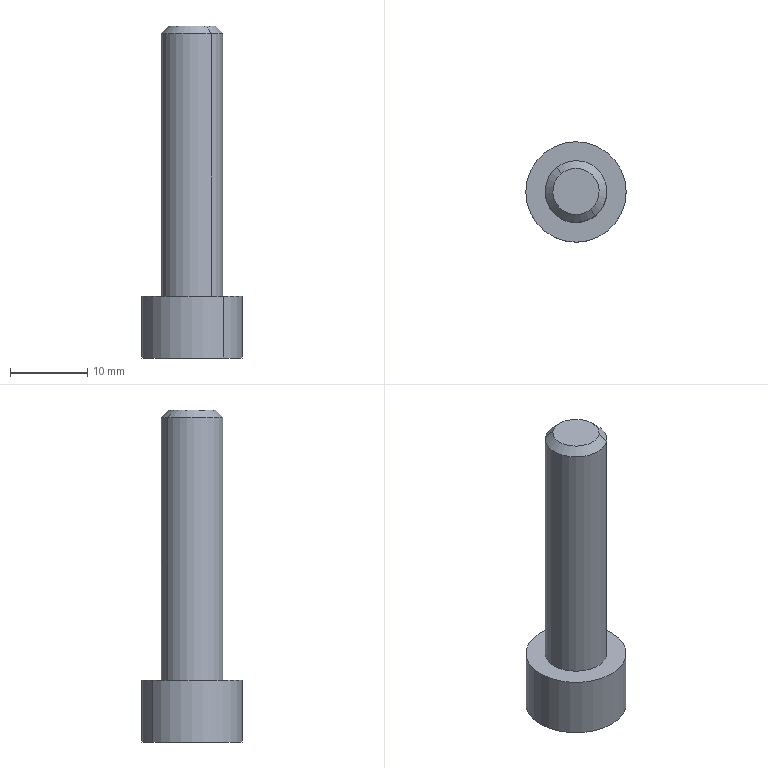Component | SolidWorks | 9HexSocketScrewM8X35-1 | 1 solid | 23 faces | box 13 x 13 x 43 mm | volume 2614 mm3 | plane 15 | cone 4 | cylinder 4 | commonest cylinder face diameters 8 x2 13 x2
STEP:
#1=CARTESIAN_POINT('',(1.263,2.918,7.047));
#2=VERTEX_POINT('',#1);
#3=CARTESIAN_POINT('',(1.411,2.734,7.047));
#4=VERTEX_POINT('',#3);
#5=CARTESIAN_POINT('',(1.337,2.826,7.047));
#6=DIRECTION('',(-0.,-0.,1.));
#7=DIRECTION('',(-0.6242,0.7813,0.));
#8=AXIS2_PLACEMENT_3D('',#5,#6,#7);
#9=CIRCLE('',#8,0.1181);
#10=EDGE_CURVE('',#2,#4,#9,.T.);
#11=ORIENTED_EDGE('',*,*,#10,.F.);
#12=CARTESIAN_POINT('',(1.239,2.949,7.008));
#13=VERTEX_POINT('',#12);
#14=CARTESIAN_POINT('',(1.263,2.918,7.047));
#15=DIRECTION('',(-0.4414,0.5524,-0.7071));
#16=VECTOR('',#15,39.37);
#17=LINE('',#14,#16);
#18=EDGE_CURVE('',#2,#13,#17,.T.);
#19=ORIENTED_EDGE('',*,*,#18,.T.);
#20=CARTESIAN_POINT('',(1.435,2.703,7.008));
#21=VERTEX_POINT('',#20);
#22=CARTESIAN_POINT('',(1.337,2.826,7.008));
#23=DIRECTION('',(0.,0.,-1.));
#24=DIRECTION('',(-0.6242,0.7813,0.));
#25=AXIS2_PLACEMENT_3D('',#22,#23,#24);
#26=CIRCLE('',#25,0.1575);
#27=EDGE_CURVE('',#21,#13,#26,.T.);
#28=ORIENTED_EDGE('',*,*,#27,.F.);
#29=CARTESIAN_POINT('',(1.411,2.734,7.047));
#30=DIRECTION('',(0.4414,-0.5524,-0.7071));
#31=VECTOR('',#30,39.37);
#32=LINE('',#29,#31);
#33=EDGE_CURVE('',#4,#21,#32,.T.);
#34=ORIENTED_EDGE('',*,*,#33,.F.);
#35=EDGE_LOOP('',(#11,#19,#28,#34));
#36=FACE_OUTER_BOUND('',#35,.T.);
#37=CARTESIAN_POINT('',(1.337,2.826,7.047));
#38=DIRECTION('',(0.,0.,-1.));
#39=DIRECTION('',(0.6242,-0.7813,0.));
#40=AXIS2_PLACEMENT_3D('',#37,#38,#39);
#41=CONICAL_SURFACE('',#40,0.1181,0.7854);
#42=ADVANCED_FACE('',(#36),#41,.T.);
#43=ORIENTED_EDGE('',*,*,#27,.T.);
#44=CARTESIAN_POINT('',(1.239,2.949,5.669));
#45=VERTEX_POINT('',#44);
#46=CARTESIAN_POINT('',(1.239,2.949,7.047));
#47=DIRECTION('',(0.,0.,-1.));
#48=VECTOR('',#47,39.37);
#49=LINE('',#46,#48);
#50=EDGE_CURVE('',#13,#45,#49,.T.);
#51=ORIENTED_EDGE('',*,*,#50,.T.);
#52=CARTESIAN_POINT('',(1.435,2.703,5.669));
#53=VERTEX_POINT('',#52);
#54=CARTESIAN_POINT('',(1.337,2.826,5.669));
#55=DIRECTION('',(-0.,-0.,1.));
#56=DIRECTION('',(-0.6242,0.7813,0.));
#57=AXIS2_PLACEMENT_3D('',#54,#55,#56);
#58=CIRCLE('',#57,0.1575);
#59=EDGE_CURVE('',#45,#53,#58,.T.);
#60=ORIENTED_EDGE('',*,*,#59,.T.);
#61=CARTESIAN_POINT('',(1.435,2.703,7.047));
#62=DIRECTION('',(0.,0.,-1.));
#63=VECTOR('',#62,39.37);
#64=LINE('',#61,#63);
#65=EDGE_CURVE('',#21,#53,#64,.T.);
#66=ORIENTED_EDGE('',*,*,#65,.F.);
#67=EDGE_LOOP('',(#43,#51,#60,#66));
#68=FACE_OUTER_BOUND('',#67,.T.);
#69=CARTESIAN_POINT('',(1.337,2.826,7.047));
#70=DIRECTION('',(0.,0.,-1.));
#71=DIRECTION('',(0.6242,-0.7813,0.));
#72=AXIS2_PLACEMENT_3D('',#69,#70,#71);
#73=CYLINDRICAL_SURFACE('',#72,0.1575);
#74=ADVANCED_FACE('',(#68),#73,.T.);
#75=CARTESIAN_POINT('',(1.337,2.826,5.591));
#76=VERTEX_POINT('',#75);
#77=CARTESIAN_POINT('',(1.423,2.718,5.512));
#78=VERTEX_POINT('',#77);
#79=CARTESIAN_POINT('',(1.423,2.718,5.512));
#80=DIRECTION('',(0.5406,-0.6766,-0.5));
#81=VECTOR('',#80,39.37);
#82=LINE('',#79,#81);
#83=EDGE_CURVE('',#76,#78,#82,.T.);
#84=ORIENTED_EDGE('',*,*,#83,.F.);
#85=CARTESIAN_POINT('',(1.251,2.933,5.512));
#86=VERTEX_POINT('',#85);
#87=CARTESIAN_POINT('',(1.251,2.933,5.512));
#88=DIRECTION('',(-0.5406,0.6766,-0.5));
#89=VECTOR('',#88,39.37);
#90=LINE('',#87,#89);
#91=EDGE_CURVE('',#76,#86,#90,.T.);
#92=ORIENTED_EDGE('',*,*,#91,.T.);
#93=CARTESIAN_POINT('',(1.316,2.962,5.512));
#94=VERTEX_POINT('',#93);
#95=CARTESIAN_POINT('',(1.337,2.826,5.512));
#96=DIRECTION('',(0.,0.,-1.));
#97=DIRECTION('',(0.6242,-0.7813,0.));
#98=AXIS2_PLACEMENT_3D('',#95,#96,#97);
#99=CIRCLE('',#98,0.1378);
#100=EDGE_CURVE('',#86,#94,#99,.T.);
#101=ORIENTED_EDGE('',*,*,#100,.T.);
#102=CARTESIAN_POINT('',(1.445,2.912,5.512));
#103=VERTEX_POINT('',#102);
#104=CARTESIAN_POINT('',(1.337,2.826,5.512));
#105=DIRECTION('',(0.,0.,-1.));
#106=DIRECTION('',(0.6242,-0.7813,0.));
#107=AXIS2_PLACEMENT_3D('',#104,#105,#106);
#108=CIRCLE('',#107,0.1378);
#109=EDGE_CURVE('',#94,#103,#108,.T.);
#110=ORIENTED_EDGE('',*,*,#109,.T.);
#111=CARTESIAN_POINT('',(1.465,2.776,5.512));
#112=VERTEX_POINT('',#111);
#113=CARTESIAN_POINT('',(1.337,2.826,5.512));
#114=DIRECTION('',(0.,0.,-1.));
#115=DIRECTION('',(0.6242,-0.7813,0.));
#116=AXIS2_PLACEMENT_3D('',#113,#114,#115);
#117=CIRCLE('',#116,0.1378);
#118=EDGE_CURVE('',#103,#112,#117,.T.);
#119=ORIENTED_EDGE('',*,*,#118,.T.);
#120=CARTESIAN_POINT('',(1.337,2.826,5.512));
#121=DIRECTION('',(0.,0.,-1.));
#122=DIRECTION('',(0.6242,-0.7813,0.));
#123=AXIS2_PLACEMENT_3D('',#120,#121,#122);
#124=CIRCLE('',#123,0.1378);
#125=EDGE_CURVE('',#112,#78,#124,.T.);
#126=ORIENTED_EDGE('',*,*,#125,.T.);
#127=EDGE_LOOP('',(#84,#92,#101,#110,#119,#126));
#128=FACE_OUTER_BOUND('',#127,.T.);
#129=CARTESIAN_POINT('',(1.337,2.826,5.512));
#130=DIRECTION('',(0.,0.,-1.));
#131=DIRECTION('',(0.6242,-0.7813,0.));
#132=AXIS2_PLACEMENT_3D('',#129,#130,#131);
#133=CONICAL_SURFACE('',#132,0.1378,1.047);
#134=ADVANCED_FACE('',(#128),#133,.F.);
#135=CARTESIAN_POINT('',(1.177,3.026,5.669));
#136=VERTEX_POINT('',#135);
#137=CARTESIAN_POINT('',(1.497,2.626,5.669));
#138=VERTEX_POINT('',#137);
#139=CARTESIAN_POINT('',(1.337,2.826,5.669));
#140=DIRECTION('',(-0.,-0.,1.));
#141=DIRECTION('',(-0.6242,0.7813,0.));
#142=AXIS2_PLACEMENT_3D('',#139,#140,#141);
#143=CIRCLE('',#142,0.2559);
#144=EDGE_CURVE('',#136,#138,#143,.T.);
#145=ORIENTED_EDGE('',*,*,#144,.F.);
#146=CARTESIAN_POINT('',(1.177,3.026,5.354));
#147=VERTEX_POINT('',#146);
#148=CARTESIAN_POINT('',(1.177,3.026,5.669));
#149=DIRECTION('',(0.,0.,-1.));
#150=VECTOR('',#149,39.37);
#151=LINE('',#148,#150);
#152=EDGE_CURVE('',#136,#147,#151,.T.);
#153=ORIENTED_EDGE('',*,*,#152,.T.);
#154=CARTESIAN_POINT('',(1.497,2.626,5.354));
#155=VERTEX_POINT('',#154);
#156=CARTESIAN_POINT('',(1.337,2.826,5.354));
#157=DIRECTION('',(-0.,-0.,1.));
#158=DIRECTION('',(-0.6242,0.7813,0.));
#159=AXIS2_PLACEMENT_3D('',#156,#157,#158);
#160=CIRCLE('',#159,0.2559);
#161=EDGE_CURVE('',#147,#155,#160,.T.);
#162=ORIENTED_EDGE('',*,*,#161,.T.);
#163=CARTESIAN_POINT('',(1.497,2.626,5.669));
#164=DIRECTION('',(0.,0.,-1.));
#165=VECTOR('',#164,39.37);
#166=LINE('',#163,#165);
#167=EDGE_CURVE('',#138,#155,#166,.T.);
#168=ORIENTED_EDGE('',*,*,#167,.F.);
#169=EDGE_LOOP('',(#145,#153,#162,#168));
#170=FACE_OUTER_BOUND('',#169,.T.);
#171=CARTESIAN_POINT('',(1.337,2.826,5.669));
#172=DIRECTION('',(0.,0.,-1.));
#173=DIRECTION('',(0.6242,-0.7813,0.));
#174=AXIS2_PLACEMENT_3D('',#171,#172,#173);
#175=CYLINDRICAL_SURFACE('',#174,0.2559);
#176=ADVANCED_FACE('',(#170),#175,.T.);
#177=CARTESIAN_POINT('',(1.358,2.69,5.512));
#178=VERTEX_POINT('',#177);
#179=CARTESIAN_POINT('',(1.229,2.74,5.512));
#180=VERTEX_POINT('',#179);
#181=CARTESIAN_POINT('',(1.337,2.826,5.512));
#182=DIRECTION('',(0.,0.,-1.));
#183=DIRECTION('',(0.6242,-0.7813,0.));
#184=AXIS2_PLACEMENT_3D('',#181,#182,#183);
#185=CIRCLE('',#184,0.1378);
#186=EDGE_CURVE('',#178,#180,#185,.T.);
#187=ORIENTED_EDGE('',*,*,#186,.F.);
#188=CARTESIAN_POINT('',(1.279,2.678,5.512));
#189=VERTEX_POINT('',#188);
#190=CARTESIAN_POINT('',(1.436,2.702,5.512));
#191=DIRECTION('',(-0.9887,-0.15,-0.));
#192=VECTOR('',#191,39.37);
#193=LINE('',#190,#192);
#194=EDGE_CURVE('',#178,#189,#193,.T.);
#195=ORIENTED_EDGE('',*,*,#194,.T.);
#196=CARTESIAN_POINT('',(1.279,2.678,5.512));
#197=DIRECTION('',(-0.6242,0.7813,-0.));
#198=VECTOR('',#197,39.37);
#199=LINE('',#196,#198);
#200=EDGE_CURVE('',#189,#180,#199,.T.);
#201=ORIENTED_EDGE('',*,*,#200,.T.);
#202=EDGE_LOOP('',(#187,#195,#201));
#203=FACE_OUTER_BOUND('',#202,.T.);
#204=CARTESIAN_POINT('',(1.337,2.826,5.512));
#205=DIRECTION('',(0.,0.,-1.));
#206=DIRECTION('',(0.6242,-0.7813,0.));
#207=AXIS2_PLACEMENT_3D('',#204,#205,#206);
#208=PLANE('',#207);
#209=ADVANCED_FACE('',(#203),#208,.T.);
#210=CARTESIAN_POINT('',(1.209,2.876,5.512));
#211=VERTEX_POINT('',#210);
#212=CARTESIAN_POINT('',(1.337,2.826,5.512));
#213=DIRECTION('',(0.,0.,-1.));
#214=DIRECTION('',(0.6242,-0.7813,0.));
#215=AXIS2_PLACEMENT_3D('',#212,#213,#214);
#216=CIRCLE('',#215,0.1378);
#217=EDGE_CURVE('',#180,#211,#216,.T.);
#218=ORIENTED_EDGE('',*,*,#217,.F.);
#219=CARTESIAN_POINT('',(1.18,2.802,5.512));
#220=VERTEX_POINT('',#219);
#221=CARTESIAN_POINT('',(1.279,2.678,5.512));
#222=DIRECTION('',(-0.6242,0.7813,-0.));
#223=VECTOR('',#222,39.37);
#224=LINE('',#221,#223);
#225=EDGE_CURVE('',#180,#220,#224,.T.);
#226=ORIENTED_EDGE('',*,*,#225,.T.);
#227=CARTESIAN_POINT('',(1.18,2.802,5.512));
#228=DIRECTION('',(0.3645,0.9312,0.));
#229=VECTOR('',#228,39.37);
#230=LINE('',#227,#229);
#231=EDGE_CURVE('',#220,#211,#230,.T.);
#232=ORIENTED_EDGE('',*,*,#231,.T.);
#233=EDGE_LOOP('',(#218,#226,#232));
#234=FACE_OUTER_BOUND('',#233,.T.);
#235=CARTESIAN_POINT('',(1.337,2.826,5.512));
#236=DIRECTION('',(0.,0.,-1.));
#237=DIRECTION('',(0.6242,-0.7813,0.));
#238=AXIS2_PLACEMENT_3D('',#235,#236,#237);
#239=PLANE('',#238);
#240=ADVANCED_FACE('',(#234),#239,.T.);
#241=CARTESIAN_POINT('',(1.337,2.826,5.512));
#242=DIRECTION('',(0.,0.,-1.));
#243=DIRECTION('',(0.6242,-0.7813,0.));
#244=AXIS2_PLACEMENT_3D('',#241,#242,#243);
#245=CIRCLE('',#244,0.1378);
#246=EDGE_CURVE('',#211,#86,#245,.T.);
#247=ORIENTED_EDGE('',*,*,#246,.F.);
#248=CARTESIAN_POINT('',(1.238,2.95,5.512));
#249=VERTEX_POINT('',#248);
#250=CARTESIAN_POINT('',(1.18,2.802,5.512));
#251=DIRECTION('',(0.3645,0.9312,0.));
#252=VECTOR('',#251,39.37);
#253=LINE('',#250,#252);
#254=EDGE_CURVE('',#211,#249,#253,.T.);
#255=ORIENTED_EDGE('',*,*,#254,.T.);
#256=CARTESIAN_POINT('',(1.238,2.95,5.512));
#257=DIRECTION('',(0.9887,0.15,0.));
#258=VECTOR('',#257,39.37);
#259=LINE('',#256,#258);
#260=EDGE_CURVE('',#249,#94,#259,.T.);
#261=ORIENTED_EDGE('',*,*,#260,.T.);
#262=ORIENTED_EDGE('',*,*,#100,.F.);
#263=EDGE_LOOP('',(#247,#255,#261,#262));
#264=FACE_OUTER_BOUND('',#263,.T.);
#265=CARTESIAN_POINT('',(1.337,2.826,5.512));
#266=DIRECTION('',(0.,0.,-1.));
#267=DIRECTION('',(0.6242,-0.7813,0.));
#268=AXIS2_PLACEMENT_3D('',#265,#266,#267);
#269=PLANE('',#268);
#270=ADVANCED_FACE('',(#264),#269,.T.);
#271=ORIENTED_EDGE('',*,*,#109,.F.);
#272=CARTESIAN_POINT('',(1.395,2.974,5.512));
#273=VERTEX_POINT('',#272);
#274=CARTESIAN_POINT('',(1.238,2.95,5.512));
#275=DIRECTION('',(0.9887,0.15,0.));
#276=VECTOR('',#275,39.37);
#277=LINE('',#274,#276);
#278=EDGE_CURVE('',#94,#273,#277,.T.);
#279=ORIENTED_EDGE('',*,*,#278,.T.);
#280=CARTESIAN_POINT('',(1.395,2.974,5.512));
#281=DIRECTION('',(0.6242,-0.7813,0.));
#282=VECTOR('',#281,39.37);
#283=LINE('',#280,#282);
#284=EDGE_CURVE('',#273,#103,#283,.T.);
#285=ORIENTED_EDGE('',*,*,#284,.T.);
#286=EDGE_LOOP('',(#271,#279,#285));
#287=FACE_OUTER_BOUND('',#286,.T.);
#288=CARTESIAN_POINT('',(1.337,2.826,5.512));
#289=DIRECTION('',(0.,0.,-1.));
#290=DIRECTION('',(0.6242,-0.7813,0.));
#291=AXIS2_PLACEMENT_3D('',#288,#289,#290);
#292=PLANE('',#291);
#293=ADVANCED_FACE('',(#287),#292,.T.);
#294=ORIENTED_EDGE('',*,*,#118,.F.);
#295=CARTESIAN_POINT('',(1.494,2.85,5.512));
#296=VERTEX_POINT('',#295);
#297=CARTESIAN_POINT('',(1.395,2.974,5.512));
#298=DIRECTION('',(0.6242,-0.7813,0.));
#299=VECTOR('',#298,39.37);
#300=LINE('',#297,#299);
#301=EDGE_CURVE('',#103,#296,#300,.T.);
#302=ORIENTED_EDGE('',*,*,#301,.T.);
#303=CARTESIAN_POINT('',(1.494,2.85,5.512));
#304=DIRECTION('',(-0.3645,-0.9312,-0.));
#305=VECTOR('',#304,39.37);
#306=LINE('',#303,#305);
#307=EDGE_CURVE('',#296,#112,#306,.T.);
#308=ORIENTED_EDGE('',*,*,#307,.T.);
#309=EDGE_LOOP('',(#294,#302,#308));
#310=FACE_OUTER_BOUND('',#309,.T.);
#311=CARTESIAN_POINT('',(1.337,2.826,5.512));
#312=DIRECTION('',(0.,0.,-1.));
#313=DIRECTION('',(0.6242,-0.7813,0.));
#314=AXIS2_PLACEMENT_3D('',#311,#312,#313);
#315=PLANE('',#314);
#316=ADVANCED_FACE('',(#310),#315,.T.);
#317=ORIENTED_EDGE('',*,*,#152,.F.);
#318=CARTESIAN_POINT('',(1.337,2.826,5.669));
#319=DIRECTION('',(-0.,-0.,1.));
#320=DIRECTION('',(-0.6242,0.7813,0.));
#321=AXIS2_PLACEMENT_3D('',#318,#319,#320);
#322=CIRCLE('',#321,0.2559);
#323=EDGE_CURVE('',#138,#136,#322,.T.);
#324=ORIENTED_EDGE('',*,*,#323,.F.);
#325=ORIENTED_EDGE('',*,*,#167,.T.);
#326=CARTESIAN_POINT('',(1.337,2.826,5.354));
#327=DIRECTION('',(-0.,-0.,1.));
#328=DIRECTION('',(-0.6242,0.7813,0.));
#329=AXIS2_PLACEMENT_3D('',#326,#327,#328);
#330=CIRCLE('',#329,0.2559);
#331=EDGE_CURVE('',#155,#147,#330,.T.);
#332=ORIENTED_EDGE('',*,*,#331,.T.);
#333=EDGE_LOOP('',(#317,#324,#325,#332));
#334=FACE_OUTER_BOUND('',#333,.T.);
#335=CARTESIAN_POINT('',(1.337,2.826,5.669));
#336=DIRECTION('',(0.,0.,-1.));
#337=DIRECTION('',(0.6242,-0.7813,0.));
#338=AXIS2_PLACEMENT_3D('',#335,#336,#337);
#339=CYLINDRICAL_SURFACE('',#338,0.2559);
#340=ADVANCED_FACE('',(#334),#339,.T.);
#341=CARTESIAN_POINT('',(1.337,2.826,5.669));
#342=DIRECTION('',(-0.,-0.,1.));
#343=DIRECTION('',(-0.6242,0.7813,0.));
#344=AXIS2_PLACEMENT_3D('',#341,#342,#343);
#345=CIRCLE('',#344,0.1575);
#346=EDGE_CURVE('',#53,#45,#345,.T.);
#347=ORIENTED_EDGE('',*,*,#346,.F.);
#348=ORIENTED_EDGE('',*,*,#59,.F.);
#349=EDGE_LOOP('',(#347,#348));
#350=FACE_BOUND('',#349,.T.);
#351=ORIENTED_EDGE('',*,*,#323,.T.);
#352=ORIENTED_EDGE('',*,*,#144,.T.);
#353=EDGE_LOOP('',(#351,#352));
#354=FACE_OUTER_BOUND('',#353,.T.);
#355=CARTESIAN_POINT('',(1.337,2.826,5.669));
#356=DIRECTION('',(-0.,-0.,1.));
#357=DIRECTION('',(-0.6242,0.7813,-0.));
#358=AXIS2_PLACEMENT_3D('',#355,#356,#357);
#359=PLANE('',#358);
#360=ADVANCED_FACE('',(#350,#354),#359,.T.);
#361=CARTESIAN_POINT('',(1.436,2.702,5.354));
#362=VERTEX_POINT('',#361);
#363=CARTESIAN_POINT('',(1.279,2.678,5.354));
#364=VERTEX_POINT('',#363);
#365=CARTESIAN_POINT('',(1.436,2.702,5.354));
#366=DIRECTION('',(-0.9887,-0.15,-0.));
#367=VECTOR('',#366,39.37);
#368=LINE('',#365,#367);
#369=EDGE_CURVE('',#362,#364,#368,.T.);
#370=ORIENTED_EDGE('',*,*,#369,.F.);
#371=CARTESIAN_POINT('',(1.494,2.85,5.354));
#372=VERTEX_POINT('',#371);
#373=CARTESIAN_POINT('',(1.494,2.85,5.354));
#374=DIRECTION('',(-0.3645,-0.9312,-0.));
#375=VECTOR('',#374,39.37);
#376=LINE('',#373,#375);
#377=EDGE_CURVE('',#372,#362,#376,.T.);
#378=ORIENTED_EDGE('',*,*,#377,.F.);
#379=CARTESIAN_POINT('',(1.395,2.974,5.354));
#380=VERTEX_POINT('',#379);
#381=CARTESIAN_POINT('',(1.395,2.974,5.354));
#382=DIRECTION('',(0.6242,-0.7813,0.));
#383=VECTOR('',#382,39.37);
#384=LINE('',#381,#383);
#385=EDGE_CURVE('',#380,#372,#384,.T.);
#386=ORIENTED_EDGE('',*,*,#385,.F.);
#387=CARTESIAN_POINT('',(1.238,2.95,5.354));
#388=VERTEX_POINT('',#387);
#389=CARTESIAN_POINT('',(1.238,2.95,5.354));
#390=DIRECTION('',(0.9887,0.15,0.));
#391=VECTOR('',#390,39.37);
#392=LINE('',#389,#391);
#393=EDGE_CURVE('',#388,#380,#392,.T.);
#394=ORIENTED_EDGE('',*,*,#393,.F.);
#395=CARTESIAN_POINT('',(1.18,2.802,5.354));
#396=VERTEX_POINT('',#395);
#397=CARTESIAN_POINT('',(1.18,2.802,5.354));
#398=DIRECTION('',(0.3645,0.9312,0.));
#399=VECTOR('',#398,39.37);
#400=LINE('',#397,#399);
#401=EDGE_CURVE('',#396,#388,#400,.T.);
#402=ORIENTED_EDGE('',*,*,#401,.F.);
#403=CARTESIAN_POINT('',(1.279,2.678,5.354));
#404=DIRECTION('',(-0.6242,0.7813,-0.));
#405=VECTOR('',#404,39.37);
#406=LINE('',#403,#405);
#407=EDGE_CURVE('',#364,#396,#406,.T.);
#408=ORIENTED_EDGE('',*,*,#407,.F.);
#409=EDGE_LOOP('',(#370,#378,#386,#394,#402,#408));
#410=FACE_BOUND('',#409,.T.);
#411=ORIENTED_EDGE('',*,*,#331,.F.);
#412=ORIENTED_EDGE('',*,*,#161,.F.);
#413=EDGE_LOOP('',(#411,#412));
#414=FACE_OUTER_BOUND('',#413,.T.);
#415=CARTESIAN_POINT('',(1.337,2.826,5.354));
#416=DIRECTION('',(-0.,-0.,1.));
#417=DIRECTION('',(-0.6242,0.7813,-0.));
#418=AXIS2_PLACEMENT_3D('',#415,#416,#417);
#419=PLANE('',#418);
#420=ADVANCED_FACE('',(#410,#414),#419,.F.);
#421=ORIENTED_EDGE('',*,*,#377,.T.);
#422=CARTESIAN_POINT('',(1.436,2.702,5.512));
#423=VERTEX_POINT('',#422);
#424=CARTESIAN_POINT('',(1.436,2.702,5.512));
#425=DIRECTION('',(0.,0.,-1.));
#426=VECTOR('',#425,39.37);
#427=LINE('',#424,#426);
#428=EDGE_CURVE('',#423,#362,#427,.T.);
#429=ORIENTED_EDGE('',*,*,#428,.F.);
#430=CARTESIAN_POINT('',(1.494,2.85,5.512));
#431=DIRECTION('',(-0.3645,-0.9312,-0.));
#432=VECTOR('',#431,39.37);
#433=LINE('',#430,#432);
#434=EDGE_CURVE('',#112,#423,#433,.T.);
#435=ORIENTED_EDGE('',*,*,#434,.F.);
#436=ORIENTED_EDGE('',*,*,#307,.F.);
#437=CARTESIAN_POINT('',(1.494,2.85,5.512));
#438=DIRECTION('',(0.,0.,-1.));
#439=VECTOR('',#438,39.37);
#440=LINE('',#437,#439);
#441=EDGE_CURVE('',#296,#372,#440,.T.);
#442=ORIENTED_EDGE('',*,*,#441,.T.);
#443=EDGE_LOOP('',(#421,#429,#435,#436,#442));
#444=FACE_OUTER_BOUND('',#443,.T.);
#445=CARTESIAN_POINT('',(1.494,2.85,5.512));
#446=DIRECTION('',(0.9312,-0.3645,0.));
#447=DIRECTION('',(0.3645,0.9312,0.));
#448=AXIS2_PLACEMENT_3D('',#445,#446,#447);
#449=PLANE('',#448);
#450=ADVANCED_FACE('',(#444),#449,.F.);
#451=ORIENTED_EDGE('',*,*,#385,.T.);
#452=ORIENTED_EDGE('',*,*,#441,.F.);
#453=ORIENTED_EDGE('',*,*,#301,.F.);
#454=ORIENTED_EDGE('',*,*,#284,.F.);
#455=CARTESIAN_POINT('',(1.395,2.974,5.512));
#456=DIRECTION('',(0.,0.,-1.));
#457=VECTOR('',#456,39.37);
#458=LINE('',#455,#457);
#459=EDGE_CURVE('',#273,#380,#458,.T.);
#460=ORIENTED_EDGE('',*,*,#459,.T.);
#461=EDGE_LOOP('',(#451,#452,#453,#454,#460));
#462=FACE_OUTER_BOUND('',#461,.T.);
#463=CARTESIAN_POINT('',(1.395,2.974,5.512));
#464=DIRECTION('',(0.7813,0.6242,0.));
#465=DIRECTION('',(-0.6242,0.7813,-0.));
#466=AXIS2_PLACEMENT_3D('',#463,#464,#465);
#467=PLANE('',#466);
#468=ADVANCED_FACE('',(#462),#467,.F.);
#469=ORIENTED_EDGE('',*,*,#393,.T.);
#470=ORIENTED_EDGE('',*,*,#459,.F.);
#471=ORIENTED_EDGE('',*,*,#278,.F.);
#472=ORIENTED_EDGE('',*,*,#260,.F.);
#473=CARTESIAN_POINT('',(1.238,2.95,5.512));
#474=DIRECTION('',(0.,0.,-1.));
#475=VECTOR('',#474,39.37);
#476=LINE('',#473,#475);
#477=EDGE_CURVE('',#249,#388,#476,.T.);
#478=ORIENTED_EDGE('',*,*,#477,.T.);
#479=EDGE_LOOP('',(#469,#470,#471,#472,#478));
#480=FACE_OUTER_BOUND('',#479,.T.);
#481=CARTESIAN_POINT('',(1.238,2.95,5.512));
#482=DIRECTION('',(-0.15,0.9887,-0.));
#483=DIRECTION('',(-0.9887,-0.15,-0.));
#484=AXIS2_PLACEMENT_3D('',#481,#482,#483);
#485=PLANE('',#484);
#486=ADVANCED_FACE('',(#480),#485,.F.);
#487=ORIENTED_EDGE('',*,*,#401,.T.);
#488=ORIENTED_EDGE('',*,*,#477,.F.);
#489=ORIENTED_EDGE('',*,*,#254,.F.);
#490=ORIENTED_EDGE('',*,*,#231,.F.);
#491=CARTESIAN_POINT('',(1.18,2.802,5.512));
#492=DIRECTION('',(0.,0.,-1.));
#493=VECTOR('',#492,39.37);
#494=LINE('',#491,#493);
#495=EDGE_CURVE('',#220,#396,#494,.T.);
#496=ORIENTED_EDGE('',*,*,#495,.T.);
#497=EDGE_LOOP('',(#487,#488,#489,#490,#496));
#498=FACE_OUTER_BOUND('',#497,.T.);
#499=CARTESIAN_POINT('',(1.18,2.802,5.512));
#500=DIRECTION('',(-0.9312,0.3645,-0.));
#501=DIRECTION('',(-0.3645,-0.9312,-0.));
#502=AXIS2_PLACEMENT_3D('',#499,#500,#501);
#503=PLANE('',#502);
#504=ADVANCED_FACE('',(#498),#503,.F.);
#505=ORIENTED_EDGE('',*,*,#407,.T.);
#506=ORIENTED_EDGE('',*,*,#495,.F.);
#507=ORIENTED_EDGE('',*,*,#225,.F.);
#508=ORIENTED_EDGE('',*,*,#200,.F.);
#509=CARTESIAN_POINT('',(1.279,2.678,5.512));
#510=DIRECTION('',(0.,0.,-1.));
#511=VECTOR('',#510,39.37);
#512=LINE('',#509,#511);
#513=EDGE_CURVE('',#189,#364,#512,.T.);
#514=ORIENTED_EDGE('',*,*,#513,.T.);
#515=EDGE_LOOP('',(#505,#506,#507,#508,#514));
#516=FACE_OUTER_BOUND('',#515,.T.);
#517=CARTESIAN_POINT('',(1.279,2.678,5.512));
#518=DIRECTION('',(-0.7813,-0.6242,-0.));
#519=DIRECTION('',(0.6242,-0.7813,0.));
#520=AXIS2_PLACEMENT_3D('',#517,#518,#519);
#521=PLANE('',#520);
#522=ADVANCED_FACE('',(#516),#521,.F.);
#523=ORIENTED_EDGE('',*,*,#369,.T.);
#524=ORIENTED_EDGE('',*,*,#513,.F.);
#525=ORIENTED_EDGE('',*,*,#194,.F.);
#526=CARTESIAN_POINT('',(1.436,2.702,5.512));
#527=DIRECTION('',(-0.9887,-0.15,-0.));
#528=VECTOR('',#527,39.37);
#529=LINE('',#526,#528);
#530=EDGE_CURVE('',#423,#178,#529,.T.);
#531=ORIENTED_EDGE('',*,*,#530,.F.);
#532=ORIENTED_EDGE('',*,*,#428,.T.);
#533=EDGE_LOOP('',(#523,#524,#525,#531,#532));
#534=FACE_OUTER_BOUND('',#533,.T.);
#535=CARTESIAN_POINT('',(1.436,2.702,5.512));
#536=DIRECTION('',(0.15,-0.9887,0.));
#537=DIRECTION('',(0.9887,0.15,0.));
#538=AXIS2_PLACEMENT_3D('',#535,#536,#537);
#539=PLANE('',#538);
#540=ADVANCED_FACE('',(#534),#539,.F.);
#541=ORIENTED_EDGE('',*,*,#125,.F.);
#542=ORIENTED_EDGE('',*,*,#434,.T.);
#543=ORIENTED_EDGE('',*,*,#530,.T.);
#544=CARTESIAN_POINT('',(1.337,2.826,5.512));
#545=DIRECTION('',(0.,0.,-1.));
#546=DIRECTION('',(0.6242,-0.7813,0.));
#547=AXIS2_PLACEMENT_3D('',#544,#545,#546);
#548=CIRCLE('',#547,0.1378);
#549=EDGE_CURVE('',#78,#178,#548,.T.);
#550=ORIENTED_EDGE('',*,*,#549,.F.);
#551=EDGE_LOOP('',(#541,#542,#543,#550));
#552=FACE_OUTER_BOUND('',#551,.T.);
#553=CARTESIAN_POINT('',(1.337,2.826,5.512));
#554=DIRECTION('',(0.,0.,-1.));
#555=DIRECTION('',(0.6242,-0.7813,0.));
#556=AXIS2_PLACEMENT_3D('',#553,#554,#555);
#557=PLANE('',#556);
#558=ADVANCED_FACE('',(#552),#557,.T.);
#559=ORIENTED_EDGE('',*,*,#91,.F.);
#560=ORIENTED_EDGE('',*,*,#83,.T.);
#561=ORIENTED_EDGE('',*,*,#549,.T.);
#562=ORIENTED_EDGE('',*,*,#186,.T.);
#563=ORIENTED_EDGE('',*,*,#217,.T.);
#564=ORIENTED_EDGE('',*,*,#246,.T.);
#565=EDGE_LOOP('',(#559,#560,#561,#562,#563,#564));
#566=FACE_OUTER_BOUND('',#565,.T.);
#567=CARTESIAN_POINT('',(1.337,2.826,5.512));
#568=DIRECTION('',(0.,0.,-1.));
#569=DIRECTION('',(0.6242,-0.7813,0.));
#570=AXIS2_PLACEMENT_3D('',#567,#568,#569);
#571=CONICAL_SURFACE('',#570,0.1378,1.047);
#572=ADVANCED_FACE('',(#566),#571,.F.);
#573=ORIENTED_EDGE('',*,*,#50,.F.);
#574=CARTESIAN_POINT('',(1.337,2.826,7.008));
#575=DIRECTION('',(0.,0.,-1.));
#576=DIRECTION('',(-0.6242,0.7813,0.));
#577=AXIS2_PLACEMENT_3D('',#574,#575,#576);
#578=CIRCLE('',#577,0.1575);
#579=EDGE_CURVE('',#13,#21,#578,.T.);
#580=ORIENTED_EDGE('',*,*,#579,.T.);
#581=ORIENTED_EDGE('',*,*,#65,.T.);
#582=ORIENTED_EDGE('',*,*,#346,.T.);
#583=EDGE_LOOP('',(#573,#580,#581,#582));
#584=FACE_OUTER_BOUND('',#583,.T.);
#585=CARTESIAN_POINT('',(1.337,2.826,7.047));
#586=DIRECTION('',(0.,0.,-1.));
#587=DIRECTION('',(0.6242,-0.7813,0.));
#588=AXIS2_PLACEMENT_3D('',#585,#586,#587);
#589=CYLINDRICAL_SURFACE('',#588,0.1575);
#590=ADVANCED_FACE('',(#584),#589,.T.);
#591=CARTESIAN_POINT('',(1.337,2.826,7.047));
#592=DIRECTION('',(-0.,-0.,1.));
#593=DIRECTION('',(-0.6242,0.7813,0.));
#594=AXIS2_PLACEMENT_3D('',#591,#592,#593);
#595=CIRCLE('',#594,0.1181);
#596=EDGE_CURVE('',#4,#2,#595,.T.);
#597=ORIENTED_EDGE('',*,*,#596,.T.);
#598=ORIENTED_EDGE('',*,*,#10,.T.);
#599=EDGE_LOOP('',(#597,#598));
#600=FACE_OUTER_BOUND('',#599,.T.);
#601=CARTESIAN_POINT('',(1.337,2.826,7.047));
#602=DIRECTION('',(-0.,-0.,1.));
#603=DIRECTION('',(-0.6242,0.7813,-0.));
#604=AXIS2_PLACEMENT_3D('',#601,#602,#603);
#605=PLANE('',#604);
#606=ADVANCED_FACE('',(#600),#605,.T.);
#607=ORIENTED_EDGE('',*,*,#18,.F.);
#608=ORIENTED_EDGE('',*,*,#596,.F.);
#609=ORIENTED_EDGE('',*,*,#33,.T.);
#610=ORIENTED_EDGE('',*,*,#579,.F.);
#611=EDGE_LOOP('',(#607,#608,#609,#610));
#612=FACE_OUTER_BOUND('',#611,.T.);
#613=CARTESIAN_POINT('',(1.337,2.826,7.047));
#614=DIRECTION('',(0.,0.,-1.));
#615=DIRECTION('',(0.6242,-0.7813,0.));
#616=AXIS2_PLACEMENT_3D('',#613,#614,#615);
#617=CONICAL_SURFACE('',#616,0.1181,0.7854);
#618=ADVANCED_FACE('',(#612),#617,.T.);
#619=CLOSED_SHELL('',(#42,#74,#134,#176,#209,#240,#270,#293,#316,#340,#360,#420,#450,#468,#486,#504,#522,#540,#558,#572,#590,#606,#618));
#620=MANIFOLD_SOLID_BREP('',#619);
#621=CARTESIAN_POINT('',(0.,0.,0.));
#622=DIRECTION('',(0.,0.,1.));
#623=DIRECTION('',(1.,0.,0.));
#624=AXIS2_PLACEMENT_3D('',#621,#622,#623);
#625=(LENGTH_UNIT()NAMED_UNIT(*)SI_UNIT($,.METRE.));
#626=LENGTH_MEASURE_WITH_UNIT(LENGTH_MEASURE(0.0254),#625);
#627=DIMENSIONAL_EXPONENTS(1.,0.,0.,0.,0.,0.,0.);
#628=(CONVERSION_BASED_UNIT('',#626)LENGTH_UNIT()NAMED_UNIT(#627));
#629=UNCERTAINTY_MEASURE_WITH_UNIT(LENGTH_MEASURE(0.00001),#628,'','');
#630=(NAMED_UNIT(*)PLANE_ANGLE_UNIT()SI_UNIT($,.RADIAN.));
#631=(NAMED_UNIT(*)SI_UNIT($,.STERADIAN.)SOLID_ANGLE_UNIT());
#632=(GEOMETRIC_REPRESENTATION_CONTEXT(3)GLOBAL_UNCERTAINTY_ASSIGNED_CONTEXT((#629))GLOBAL_UNIT_ASSIGNED_CONTEXT((#628,#630,#631))REPRESENTATION_CONTEXT('',''));
#633=ADVANCED_BREP_SHAPE_REPRESENTATION('',(#620,#624),#632);
#634=COLOUR_RGB('',0.7922,0.8196,0.9333);
#635=FILL_AREA_STYLE_COLOUR('',#634);
#636=FILL_AREA_STYLE('',(#635));
#637=SURFACE_STYLE_FILL_AREA(#636);
#638=SURFACE_SIDE_STYLE('',(#637));
#639=SURFACE_STYLE_USAGE(.BOTH.,#638);
#640=PRESENTATION_STYLE_ASSIGNMENT((#639));
#641=STYLED_ITEM('',(#640),#620);
#642=PRESENTATION_LAYER_ASSIGNMENT('','',(#641));
#643=(LENGTH_UNIT()NAMED_UNIT(*)SI_UNIT($,.METRE.));
#644=LENGTH_MEASURE_WITH_UNIT(LENGTH_MEASURE(0.0254),#643);
#645=DIMENSIONAL_EXPONENTS(1.,0.,0.,0.,0.,0.,0.);
#646=(CONVERSION_BASED_UNIT('',#644)LENGTH_UNIT()NAMED_UNIT(#645));
#647=UNCERTAINTY_MEASURE_WITH_UNIT(LENGTH_MEASURE(0.00001),#646,'','');
#648=(NAMED_UNIT(*)PLANE_ANGLE_UNIT()SI_UNIT($,.RADIAN.));
#649=(NAMED_UNIT(*)SI_UNIT($,.STERADIAN.)SOLID_ANGLE_UNIT());
#650=(GEOMETRIC_REPRESENTATION_CONTEXT(3)GLOBAL_UNCERTAINTY_ASSIGNED_CONTEXT((#647))GLOBAL_UNIT_ASSIGNED_CONTEXT((#646,#648,#649))REPRESENTATION_CONTEXT('',''));
#651=MECHANICAL_DESIGN_GEOMETRIC_PRESENTATION_REPRESENTATION('',(#641),#650);